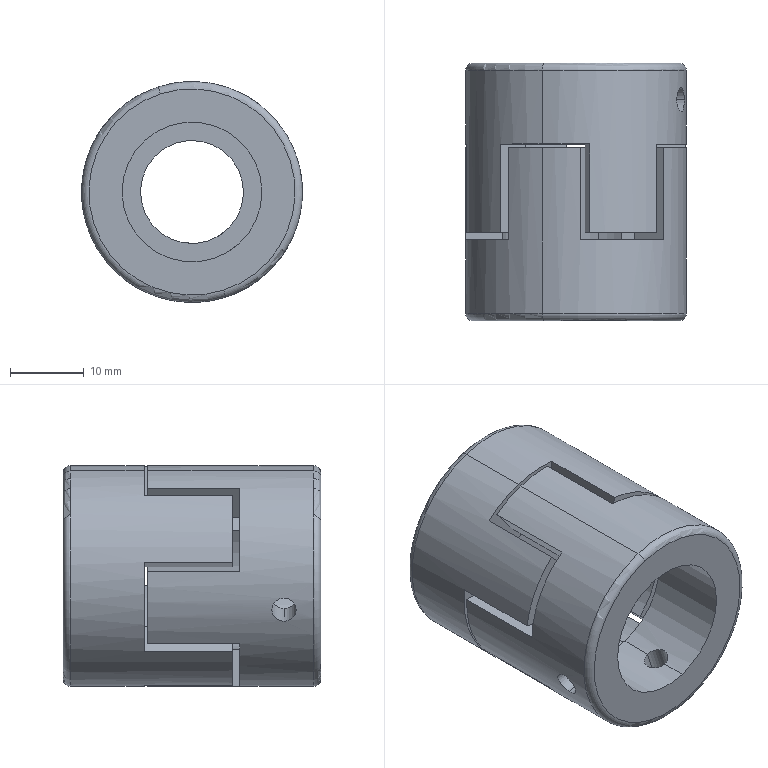Component | SolidWorks | Coupling_XF5-30-14-10-1 | 2 solids | 57 faces | volume 14743 mm3 | plane 28 | cylinder 25 | torus 4 | commonest cylinder face diameters 20 x9 3.3 x8 30 x4 14 x2 19 x2